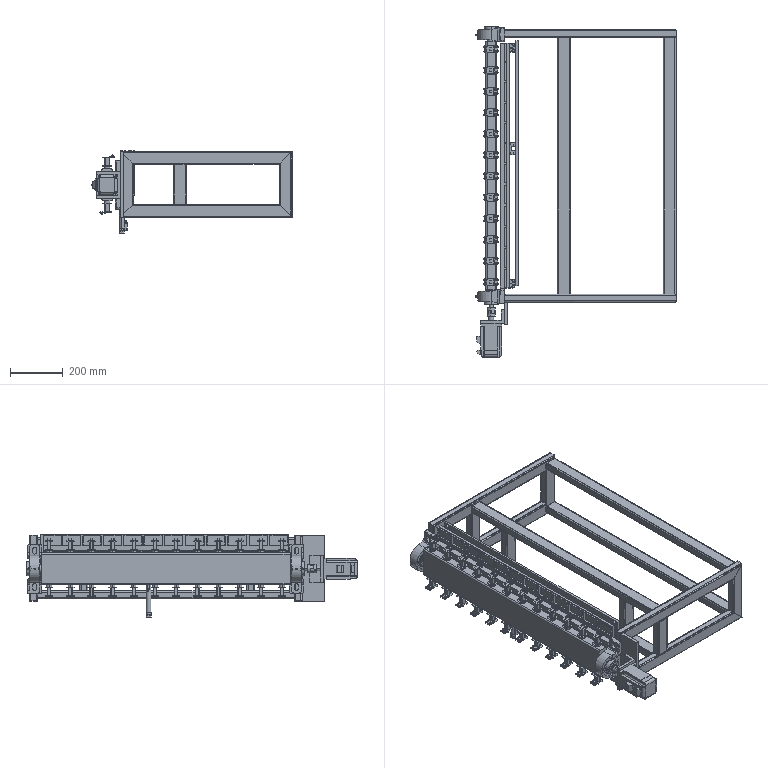Assembly | SolidWorks | mm | 79 component files | 102 solids | 4838 faces | box 758 x 1248.45 x 310 mm | volume 12114477 mm3 | plane 3719 | cylinder 933 | cone 142 | torus 38 | sphere 4 | spline 2 | commonest cylinder face diameters 10 x118 20 x117 1.5 x96 1 x96 10.4 x64 5.2 x64 4 x48 3.08 x40
Bill of materials:
750WServoMotor(ML)A | 1 |  | Rectangular prismatic body with a square end flange, four corner through-holes, a round boss and a cylindrical shaft sticking out of the flange face. Small block on one side near the back end. Rounded edges at the rear.
CoilSleeveFixingRod | 24 | Plain Carbon Steel | Short solid cylinder with a square-section prism rising coaxially from one end face.
Coupling_XF5-30-14-10 | 1 |  | Cylindrical sleeve with a central through-bore. A stepped, interlocking slit pattern cuts through the wall around the middle. Small radial holes sit near both ends.
Cylinder | 1 | Plain Carbon Steel | Long slender cylindrical tube with polygonal end caps. A short stepped stub sticks out of one end, and two small rectangular blocks with small cylindrical pins are mounted on the sides, one near each end.
FlipAxis | 1 | Plain Carbon Steel | Solid stepped cylindrical pin with three coaxial diameters: a large short head, a long middle body and a smaller-diameter end.
FlipAxisOne | 1 | Plain Carbon Steel | Solid cylinder with a short, larger-diameter head at one end, forming a headed pin shape.
FlipMechanismFixingBracket | 1 |  | Open rectangular frame built from square-section bars: two end frames joined by long longitudinal rails, with intermediate vertical posts and a cross member.
FlipMotorSupportPlate | 1 | Plain Carbon Steel | Plain thin rectangular plate.
FlipSolderPlate | 1 | Plain Carbon Steel | Long rectangular bar with a row of evenly spaced holes along one face and a large hole in the end face, along the bar's length.
LYB-0170 | 1 |  | Bracket with a flat tab that has a rounded end and one large through-hole. The tab joins a block with a U-shaped cutout, made up of two upright pillars, each with two through-holes.
RosinBox | 12 | Plain Carbon Steel | Plain rectangular block or plate of moderate thickness.
RotatingBearingHousing | 2 | Plain Carbon Steel | Flange-type housing with a rounded body holding a cylindrical insert with a central bore, and a straight mounting flange with two slotted holes. A small nipple-like projection sticks out of the rounded side.
RotatingMotorFixingPlate | 1 | Plain Carbon Steel | L-shaped (angle) bracket of constant thickness: two flat legs at roughly 90 degrees, with one large circular through-hole in one leg.
SolderBox | 1 | Plain Carbon Steel | Long straight bar with a solid rectangular cross-section and plain square-cut ends.
SolderBoxFixingBracket | 1 | Plain Carbon Steel | Thin flat rectangular strip or plate: long and fairly narrow, with very small thickness and no visible features.
SolderBoxFixingBracketOne | 1 | Plain Carbon Steel | Thin flat rectangular strip or plate with no visible features. Its proportions are very close to unnamed part, and it looks slightly wider relative to its length.
block_SXRB24 | 2 |  | Rectangular prismatic block with a C-shaped cross-section: a wide open channel runs the full length of one side, with rounded relief grooves at the channel corners. It has small shallow steps along the outer side faces, chamfered corners, a small conical or domed pin on the top face, and two circular markings with a cross inside on the top face.
LinearGuide | 2 |  | Long slender prismatic bar. Its constant cross-section has two opposed large semicircular notches, and two corners are chamfered. Three small round through-holes are evenly spaced along one long face.
WindingFrame | 24 | ABS PC | Spool- or bobbin-like body: a hollow tube with a rectangular inside opening joins two flat end flanges, each with rounded corners on one end. One flange has an extended stepped block carrying two thin protruding pins and a flat tab with a small round hole.
Mates:
1. concentric | FlipSolderPlate-1 face at (-864.885, -367.907, 975.102) dir (0, 0, 1) r 10 | CoilSleeveFixingRod-1 face at (-864.885, -367.907, 1105.102) dir (0, 0, -1) r 10
2. distance | CoilSleeveFixingRod-1 face at (-864.885, -367.907, 1085.102) dir (0, 0, -1) | FlipSolderPlate-1 face at (-884.885, 542.093, 1095.102) dir (0, 0, 1)
3. concentric | FlipSolderPlate-1 face at (-864.885, -397.907, 1035.102) dir (0, 1, 0) r 15 | FlipAxis-4 face at (-864.885, -407.907, 1035.102) dir (0, 1, 0) r 15
4. coincident | FlipSolderPlate-1 face at (-884.885, -397.907, 1095.102) dir (0, -1, 0) | FlipAxis-4 face at (-864.885, -397.907, 1035.102) dir (0, 1, 0)
5. concentric | FlipSolderPlate-1 face at (-864.885, -397.907, 1035.102) dir (0, 1, 0) r 15 | FlipAxisOne-4 face at (-864.885, 552.093, 1035.102) dir (0, -1, 0) r 15
6. coincident | FlipSolderPlate-1 face at (-884.885, 542.093, 975.102) dir (0, 1, 0) | FlipAxisOne-4 face at (-864.885, 542.093, 1035.102) dir (0, -1, 0)
7. concentric | FlipAxis-4 face at (-864.885, -452.907, 1035.102) dir (0, 1, 0) r 12.5 | RotatingBearingHousing-1 face at (-864.885, -508.926, 1035.102) dir (0, 1, 0) r 12.5
8. parallel | FlipSolderPlate-1 face at (-884.885, 76.501, 940) dir (-1, 0, 0) | RotatingBearingHousing-1 face at (-815.685, -449.157, 943.102) dir (1, 0, 0)
9. coincident | FlipAxis-4 face at (-864.885, -407.907, 1035.102) dir (0, -1, 0) | RotatingBearingHousing-1 face at (-864.885, -407.907, 1035.102) dir (0, 1, 0)
10. concentric | FlipAxisOne-4 face at (-864.885, 594.093, 1035.102) dir (0, -1, 0) r 12.5 | RotatingBearingHousing-2 face at (-864.885, 653.111, 1035.102) dir (0, -1, 0) r 12.5
11. coincident | FlipAxisOne-4 face at (-864.885, 552.093, 1035.102) dir (0, 1, 0) | RotatingBearingHousing-2 face at (-864.885, 552.093, 1035.102) dir (0, -1, 0)
12. concentric | Coupling_XF5-30-14-10-1 face at (-864.885, -497.907, 1035.102) dir (0, 1, 0) r 9.5 | 750WServoMotor(ML)A-1 face at (-864.885, -489.907, 1035.102) dir (0, -1, 0) r 9.5
13. distance | 750WServoMotor(ML)A-1 face at (-864.885, -489.907, 1035.102) dir (0, 1, 0) | Coupling_XF5-30-14-10-1 face at (-864.885, -497.907, 1035.102) dir (0, -1, 0)
14. concentric | 750WServoMotor(ML)A-1 face at (-864.885, -521.907, 1035.102) dir (0, -1, 0) r 35 | RotatingMotorFixingPlate-1 face at (-864.885, -524.907, 1035.102) dir (0, 1, 0) r 35
15. coincident | 750WServoMotor(ML)A-1 face at (-864.885, -524.907, 1035.102) dir (0, 1, 0) | RotatingMotorFixingPlate-1 face at (-860.285, -524.907, 1035.102) dir (0, -1, 0)
16. parallel | RotatingBearingHousing-2 face at (-815.685, 593.343, 1127.102) dir (1, 0, 0) | RotatingMotorFixingPlate-1 face at (-815.685, -512.907, 985.102) dir (1, 0, 0)
17. coincident | 750WServoMotor(ML)A-1 face at (-904.885, -624.907, 1075.102) dir (-1, 0, 0) | RotatingMotorFixingPlate-1 face at (-904.885, -512.907, 985.102) dir (-1, 0, 0)
18. parallel | FlipSolderPlate-1 face at (-884.885, 76.501, 940) dir (-1, 0, 0) | RotatingBearingHousing-2 face at (-815.685, 593.343, 1127.102) dir (1, 0, 0)
19. parallel | FlipSolderPlate-1 face at (-884.885, 76.501, 940) dir (-1, 0, 0) | CoilSleeveFixingRod-1 face at (-872.135, -373.157, 1139.102) dir (-1, 0, 0)
20. coincident | CoilSleeveFixingRod-24 face at (-857.635, -362.657, 931.102) dir (0, 1, 0) | WindingFrame-1 face at (-872.135, -362.657, 965.102) dir (0, -1, 0)
21. coincident | CoilSleeveFixingRod-24 face at (-872.135, -362.657, 931.102) dir (-1, 0, 0) | WindingFrame-1 face at (-872.135, -362.657, 965.102) dir (1, 0, 0)
22. coincident | CoilSleeveFixingRod-24 face at (-874.885, -367.907, 965.102) dir (0, 0, -1) | WindingFrame-1 face at (-864.885, -367.907, 965.102) dir (0, 0, 1)
23. coincident | CoilSleeveFixingRod-1 face at (-872.135, -362.657, 1139.102) dir (0, 1, 0) | WindingFrame-13 face at (-857.635, -362.657, 1105.102) dir (0, -1, 0)
24. coincident | CoilSleeveFixingRod-1 face at (-857.635, -362.657, 1139.102) dir (1, 0, 0) | WindingFrame-13 face at (-857.635, -362.657, 1105.102) dir (-1, 0, 0)
25. coincident | CoilSleeveFixingRod-1 face at (-854.885, -367.907, 1105.102) dir (0, 0, 1) | WindingFrame-13 face at (-864.885, -367.907, 1105.102) dir (0, 0, -1)
26. distance | SolderBoxFixingBracket-1 face at (-796.135, -390.407, 1013.102) dir (0, -1, 0) | WindingFrame-13 face at (-853.135, -380.407, 1141.102) dir (0, -1, 0)
27. distance | SolderBoxFixingBracket-1 face at (-806.135, 72.093, 1088.102) dir (-1, 0, 0) | WindingFrame-13 face at (-836.135, -367.907, 1140.402) dir (1, 0, 0)
28. distance | SolderBoxFixingBracket-1 face at (-796.135, 534.593, 1163.102) dir (0, 0, 1) | WindingFrame-13 face at (-864.885, -367.907, 1143.102) dir (0, 0, 1)
29. coincident | SolderBoxFixingBracket-1 face at (-796.135, 72.093, 1088.102) dir (1, 0, 0) | SXRZ24_280-1/block_SXRB24-2 face at (-796.135, -382.407, 1091.877) dir (-1, 0, 0)
30. coincident | SolderBoxFixingBracket-1 face at (-796.135, -390.407, 1013.102) dir (0, -1, 0) | SXRZ24_280-1/block_SXRB24-2 face at (-795.145, -390.407, 1091.877) dir (0, -1, 0)
31. coincident | SolderBoxFixingBracket-1 face at (-796.135, 72.093, 1088.102) dir (1, 0, 0) | SXRZ24_280-2/block_SXRB24-2 face at (-796.135, 508.593, 1091.877) dir (-1, 0, 0)
32. coincident | SolderBoxFixingBracket-1 face at (-796.135, 534.593, 1013.102) dir (0, 1, 0) | SXRZ24_280-2/block_SXRB24-2 face at (-786.135, 534.593, 1091.877) dir (0, 1, 0)
33. coincident | SXRZ24_280-1/LinearGuide-1 face at (-772.135, -524.635, 1163.102) dir (0, 0, 1) | SXRZ24_280-2/LinearGuide-1 face at (-772.135, 366.365, 1163.102) dir (0, 0, 1)
34. coincident | SolderBoxFixingBracket-1 face at (-796.135, 534.593, 1163.102) dir (0, 0, 1) | SXRZ24_280-1/LinearGuide-1 face at (-772.135, -524.635, 1163.102) dir (0, 0, 1)
35. coincident | SXRZ24_280-1/LinearGuide-1 face at (-772.135, -380.907, 1223.102) dir (1, 0, 0) | SolderBoxFixingBracketOne-2 face at (-772.135, 81.593, 1078.102) dir (-1, 0, 0)
36. coincident | SXRZ24_280-1/LinearGuide-1 face at (-777.24, -380.907, 1223.102) dir (0, -1, 0) | SolderBoxFixingBracketOne-2 face at (-762.135, -380.907, 993.102) dir (0, -1, 0)
37. coincident | SXRZ24_280-1/LinearGuide-1 face at (-772.135, -524.635, 1163.102) dir (0, 0, 1) | SolderBoxFixingBracketOne-2 face at (-762.135, 544.093, 1163.102) dir (0, 0, 1)
38. coincident | SolderBoxFixingBracketOne-2 face at (-762.135, 544.093, 993.102) dir (0, 0, -1) | LYB-0170-1 face at (-782.135, 158.514, 993.102) dir (0, 0, -1)
39. concentric | Cylinder-1 face at (-810.135, 136.014, 1008.102) dir (0, 0, -1) r 5 | LYB-0170-1 face at (-810.135, 136.014, 1003.102) dir (0, 0, 1) r 5.5
40. coincident | Cylinder-1 face at (-810.135, 136.014, 1000.102) dir (0, 0, 1) | LYB-0170-1 face at (-793.635, 158.514, 1000.102) dir (0, 0, -1)
41. coincident | SolderBoxFixingBracket-1 face at (-806.135, 72.093, 1088.102) dir (-1, 0, 0) | RosinBox-1 face at (-806.135, -355.407, 1143.102) dir (1, 0, 0)
42. coincident | SolderBoxFixingBracket-1 face at (-796.135, 534.593, 1163.102) dir (0, 0, 1) | RosinBox-1 face at (-814.135, -390.407, 1163.102) dir (0, 0, 1)
43. coincident | SolderBoxFixingBracket-1 face at (-796.135, -390.407, 1013.102) dir (0, -1, 0) | RosinBox-1 face at (-814.135, -390.407, 1123.102) dir (0, -1, 0)
44. coincident | SolderBoxFixingBracket-1 face at (-806.135, 72.093, 1088.102) dir (-1, 0, 0) | RosinBox-2 face at (-806.135, -278.157, 1143.102) dir (1, 0, 0)
45. coincident | SolderBoxFixingBracket-1 face at (-796.135, 534.593, 1163.102) dir (0, 0, 1) | RosinBox-2 face at (-814.135, -313.157, 1163.102) dir (0, 0, 1)
46. distance | WindingFrame-14 edge at (-857.635, -293.157, 1139.102) dir (-1, 0, 0) | RosinBox-2 face at (-814.135, -313.157, 1123.102) dir (0, -1, 0)
47. coincident | SolderBoxFixingBracket-1 face at (-796.135, 534.593, 1013.102) dir (0, 1, 0) | RosinBox-13 face at (-814.135, 534.593, 1123.102) dir (0, 1, 0)
48. coincident | SolderBoxFixingBracket-1 face at (-806.135, 72.093, 1088.102) dir (-1, 0, 0) | RosinBox-13 face at (-806.135, 499.593, 1143.102) dir (1, 0, 0)
49. coincident | SolderBoxFixingBracket-1 face at (-796.135, 534.593, 1163.102) dir (0, 0, 1) | RosinBox-13 face at (-814.135, 464.593, 1163.102) dir (0, 0, 1)
50. coincident | SolderBoxFixingBracket-1 face at (-806.135, 72.093, 1088.102) dir (-1, 0, 0) | SolderBox-1 face at (-806.135, 72.093, 1073.102) dir (1, 0, 0)
51. coincident | SolderBoxFixingBracket-1 face at (-796.135, 534.593, 1013.102) dir (0, 1, 0) | SolderBox-1 face at (-831.135, 534.593, 1043.102) dir (0, 1, 0)
52. distance | SolderBox-1 face at (-831.135, -390.407, 1103.102) dir (0, 0, 1) | RosinBox-10 face at (-814.135, 314.843, 1123.102) dir (0, 0, -1)
53. coincident | RotatingBearingHousing-1 face at (-815.685, -449.157, 943.102) dir (1, 0, 0) | FlipMechanismFixingBracket-1 face at (-815.685, -419.357, 1137.102) dir (-1, 0, 0)
54. distance | RotatingBearingHousing-1 face at (-815.685, -449.157, 1035.102) dir (0, -1, 0) | FlipMechanismFixingBracket-1 face at (-770.885, -444.157, 1137.102) dir (0, -1, 0)
55. distance | RotatingBearingHousing-1 face at (-815.685, -449.157, 1127.102) dir (0, 0, 1) | FlipMechanismFixingBracket-1 face at (-190.685, -419.357, 1162.102) dir (0, 0, 1)
56. coincident | RotatingMotorFixingPlate-1 face at (-815.685, -512.907, 985.102) dir (1, 0, 0) | FlipMotorSupportPlate-1 face at (-815.685, -486.157, 1037.102) dir (-1, 0, 0)
57. concentric | FlipAxis-4 face at (-864.885, -470.907, 1035.102) dir (0, 1, 0) r 7 | Coupling_XF5-30-14-10-1 face at (-864.885, -462.907, 1035.102) dir (0, -1, 0) r 7
58. distance | Coupling_XF5-30-14-10-1 face at (-864.885, -462.907, 1035.102) dir (0, 1, 0) | FlipAxis-4 face at (-864.885, -470.907, 1035.102) dir (0, -1, 0)
59. coincident | FlipMechanismFixingBracket-1 face at (-190.685, -419.357, 1162.102) dir (0, 0, 1) | FlipMotorSupportPlate-1 face at (-803.685, -528.157, 1162.102) dir (0, 0, 1)
60. coincident | FlipMechanismFixingBracket-1 face at (-770.885, -444.157, 1137.102) dir (0, -1, 0) | FlipMotorSupportPlate-1 face at (-803.685, -444.157, 912.102) dir (0, 1, 0)
61. coincident | SolderBoxFixingBracketOne-2 face at (-772.135, 81.593, 1078.102) dir (-1, 0, 0) | LYB-0170-1 face at (-772.135, 158.514, 993.102) dir (1, 0, 0)
62. concentric | LinearGuide-1 face at (-7.5, 7.305, 140) dir (0, 0, -1) r 2.2 | block_SXRB24-2 face at (-7.5, 7.305, 8.775) dir (0, 0, -1) r 2.2
63. concentric | LinearGuide-1 face at (7.5, 7.305, 140) dir (0, 0, -1) r 2.2 | block_SXRB24-2 face at (7.5, 7.305, 8.775) dir (0, 0, -1) r 2.2